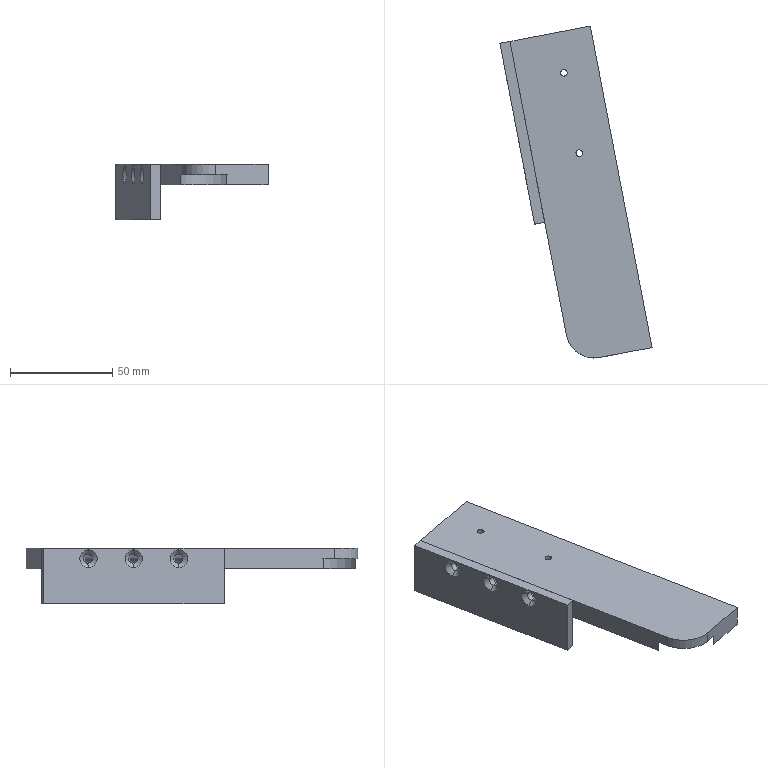Component | SolidWorks | OuterBandCylinderFixingPlate-1 | 2 solids | 43 faces | box 74.36 x 162.28 x 27 mm | volume 71082 mm3 | cylinder 18 | plane 13 | cone 12 | commonest cylinder face diameters 4.5 x12 3.3 x4 30 x1 28 x1
build123d program:
from build123d import *

# Parameters (mm, degrees)
BOSS_EXTRUDE1_DEPTH                         = 5
BOSS_EXTRUDE2_DEPTH                         = 5
M4_TAPPED_HOLE2_D                           = 3.3
SKETCH8_W                                   = 5
SKETCH8_H                                   = 90
BOSS_EXTRUDE3_DEPTH                         = 27
SPLIT1_SURFACE_1_BACK                       = 169.386
SPLIT1_SURFACE_1_DEPTH                      = 338.772
SPLIT1_SURFACE_2_BACK                       = 169.386
SPLIT1_SURFACE_2_DEPTH                      = 338.772
M4_PHILLIPS_RAISED_COUNTERSUNK_WOOD_2_COUNT = 2
M4_PHILLIPS_RAISED_COUNTERSUNK_WOOD_2_PITCH = 45
M4_PHILLIPS_RAISED_COUNTERSUNK_WOOD_3_COUNT = 2
M4_PHILLIPS_RAISED_COUNTERSUNK_WOOD_3_PITCH = 22.5


with BuildPart() as part:
    # Sketch2_4 → Boss-Extrude1 (new body)
    with BuildSketch(Plane.XY):
        with BuildLine():
            Line((0, 14), (-26, 14))
            Line((-26, 14), (-26, -146))
            Line((-26, -146), (14, -146))
            Line((14, -146), (14, 0))
            ThreePointArc((14, 0), (9.899, 9.899), (0, 14))
        make_face()
    extrude(amount=BOSS_EXTRUDE1_DEPTH)

    # Sketch2_4 2 → Boss-Extrude2 (add)
    with BuildSketch(Plane.XY):
        with BuildLine():
            ThreePointArc((14, -5.385), (-10.607, -10.607), (-5.385, 14))
            Line((-5.385, 14), (-26, 14))
            Line((-26, 14), (-26, -146))
            Line((-26, -146), (14, -146))
            Line((14, -146), (14, -5.385))
        make_face()
    extrude(amount=-BOSS_EXTRUDE2_DEPTH)

    # M4 Tapped Hole2 (through all)
    with Locations(Plane(origin=(0, 0, -5), x_dir=(-1, 0, 0), z_dir=(0, 0, -1))):
        with Locations((9, -86), (9, -126)):
            Hole(M4_TAPPED_HOLE2_D / 2)

    # Sketch8 → Boss-Extrude3 (add)
    with BuildSketch(Plane.XY.offset(5)):
        with Locations((16.5, -101)):
            Rectangle(SKETCH8_W, SKETCH8_H)
    extrude(amount=-BOSS_EXTRUDE3_DEPTH)


with BuildPart() as body_2:
    # Split1: the piece behind the surface
    add(part.part)
    # Split1 surface: a surface, the sketch's curves swept straight by 338.772 mm
    with BuildLine(Plane.XY.offset(5).offset(-SPLIT1_SURFACE_1_BACK), mode=Mode.PRIVATE) as split1_surface_1_path:
        Line((14, -56), (14, -146))
    split1_surface_1 = Shell.extrude(split1_surface_1_path.wire(), (0 * SPLIT1_SURFACE_1_DEPTH, 0 * SPLIT1_SURFACE_1_DEPTH, 1 * SPLIT1_SURFACE_1_DEPTH))
    split(bisect_by=split1_surface_1, keep=Keep.BOTTOM)


with BuildPart() as part_1:
    add(part.part)

    # Split1: split by a surface, the side it looks to stays
    # Split1 surface: a surface, the sketch's curves swept straight by 338.772 mm
    with BuildLine(Plane.XY.offset(5).offset(-SPLIT1_SURFACE_2_BACK), mode=Mode.PRIVATE) as split1_surface_2_path:
        Line((14, -56), (14, -146))
    split1_surface_2 = Shell.extrude(split1_surface_2_path.wire(), (0 * SPLIT1_SURFACE_2_DEPTH, 0 * SPLIT1_SURFACE_2_DEPTH, 1 * SPLIT1_SURFACE_2_DEPTH))
    split(bisect_by=split1_surface_2, keep=Keep.TOP)


with BuildPart() as m4_phillips_raised_countersunk_wood_scre_tool:
    # Sketch14 → M4 Phillips Raised Countersunk Wood Scre (revolve)
    with BuildSketch(Plane(origin=(19, -123.5, 0), x_dir=(0, 0, -1), z_dir=(0, 1, 0))):
        Polygon((0, 0), (0, 21.352), (2.25, 20), (2.25, 2.05), (4.3, 0), align=None)
    m4_phillips_raised_countersunk_wood_scre = revolve(axis=Axis((25.35, -123.5, 0), (-1, 0, 0)))


with BuildPart() as part_2:
    add(part_1.part)

    # M4 Phillips Raised Countersunk Wood Scre: cut by m4_phillips_raised_countersunk_wood_scre_tool
    add(m4_phillips_raised_countersunk_wood_scre_tool.part, mode=Mode.SUBTRACT)


with BuildPart() as body_2_1:
    add(body_2.part)

    # M4 Phillips Raised Countersunk Wood Scre: cut by m4_phillips_raised_countersunk_wood_scre_tool
    add(m4_phillips_raised_countersunk_wood_scre_tool.part, mode=Mode.SUBTRACT)


with BuildPart() as m4_phillips_raised_countersunk_wood_2_tool:
    # M4 Phillips Raised Countersunk Wood  2: M4 Phillips Raised Countersunk Wood Scre ×2
    with Locations(*[(0, i * M4_PHILLIPS_RAISED_COUNTERSUNK_WOOD_2_PITCH, 0) for i in range(1, M4_PHILLIPS_RAISED_COUNTERSUNK_WOOD_2_COUNT)]):
        add(m4_phillips_raised_countersunk_wood_scre)


with BuildPart() as part_3:
    add(part_2.part)

    # M4 Phillips Raised Countersunk Wood  2: cut by m4_phillips_raised_countersunk_wood_2_tool
    add(m4_phillips_raised_countersunk_wood_2_tool.part, mode=Mode.SUBTRACT)


with BuildPart() as body_2_2:
    add(body_2_1.part)

    # M4 Phillips Raised Countersunk Wood  2: cut by m4_phillips_raised_countersunk_wood_2_tool
    add(m4_phillips_raised_countersunk_wood_2_tool.part, mode=Mode.SUBTRACT)


with BuildPart() as m4_phillips_raised_countersunk_wood_3_tool:
    # M4 Phillips Raised Countersunk Wood  3: M4 Phillips Raised Countersunk Wood Scre ×2
    with Locations(*[(0, i * M4_PHILLIPS_RAISED_COUNTERSUNK_WOOD_3_PITCH, 0) for i in range(1, M4_PHILLIPS_RAISED_COUNTERSUNK_WOOD_3_COUNT)]):
        add(m4_phillips_raised_countersunk_wood_scre)


with BuildPart() as part_4:
    add(part_3.part)

    # M4 Phillips Raised Countersunk Wood  3: cut by m4_phillips_raised_countersunk_wood_3_tool
    add(m4_phillips_raised_countersunk_wood_3_tool.part, mode=Mode.SUBTRACT)


with BuildPart() as body_2_3:
    add(body_2_2.part)

    # M4 Phillips Raised Countersunk Wood  3: cut by m4_phillips_raised_countersunk_wood_3_tool
    add(m4_phillips_raised_countersunk_wood_3_tool.part, mode=Mode.SUBTRACT)


solid = Compound([part_4.part, body_2_3.part])

# Placed as in the assembly
solid = solid.moved(Location((-331.696, -83.151, 364.468), (0, 0, -169.133)))